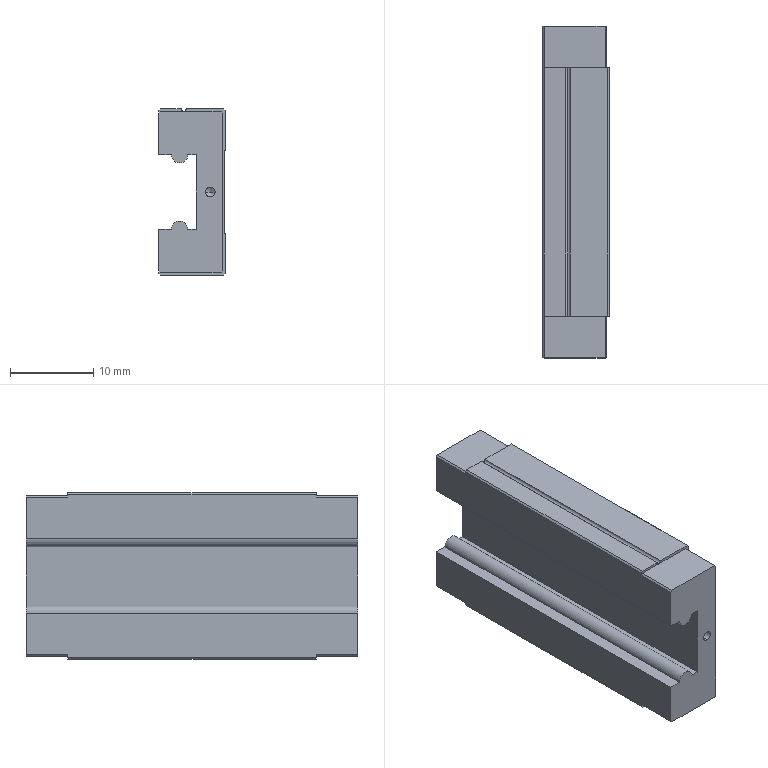Component | SolidWorks | MGN9-HSlider-D-1 | 1 solid | 67 faces | volume 4630 mm3 | plane 38 | cylinder 17 | cone 12 | commonest cylinder face diameters 3 x8 1.2 x4 2 x3 0.6 x2 | material 45